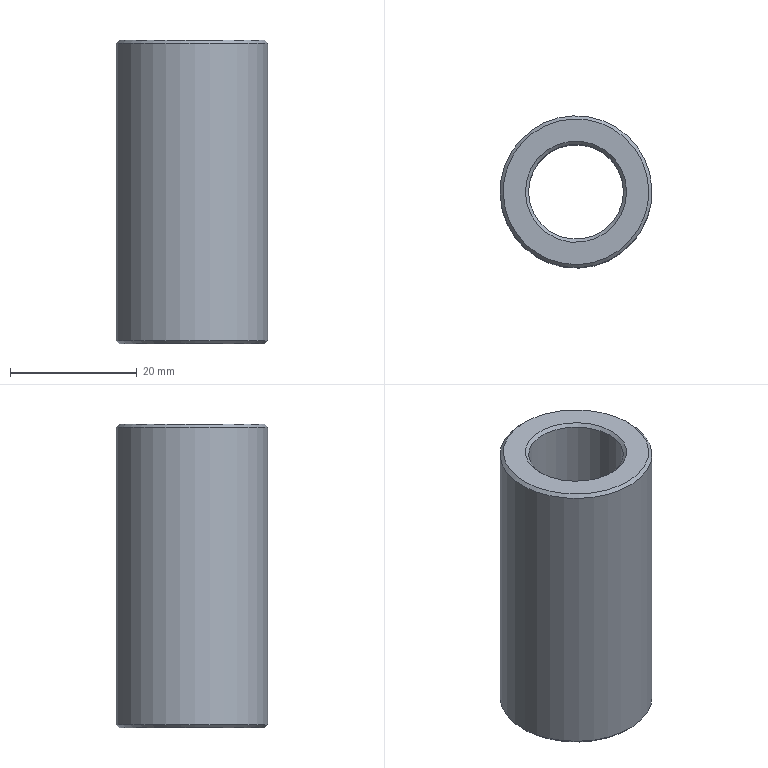Component | NX | BUSHING | 1 solid | 8 faces | box 24 x 24 x 48 mm | volume 13202 mm3 | cone 4 | cylinder 2 | plane 2 | commonest cylinder face diameters 24 x1 15 x1
STEP:
#1=CARTESIAN_POINT('',(0.,0.,0.));
#2=DIRECTION('',(0.,0.,1.));
#3=DIRECTION('',(1.,0.,0.));
#4=AXIS2_PLACEMENT_3D('',#1,#2,#3);
#5=CARTESIAN_POINT('',(-39.104,-11.276,75.5));
#6=VERTEX_POINT('',#5);
#7=CARTESIAN_POINT('',(-35.,0.,75.5));
#8=DIRECTION('',(0.,0.,1.));
#9=DIRECTION('',(-0.342,-0.9397,0.));
#10=AXIS2_PLACEMENT_3D('',#7,#8,#9);
#11=CIRCLE('',#10,12.);
#12=CARTESIAN_POINT('',(-35.,0.,123.));
#13=DIRECTION('',(0.,0.,-1.));
#14=DIRECTION('',(-0.342,-0.9397,0.));
#15=AXIS2_PLACEMENT_3D('',#12,#13,#14);
#16=CYLINDRICAL_SURFACE('',#15,12.);
#17=CARTESIAN_POINT('',(6.283,47.5));
#18=DIRECTION('',(-1.,0.));
#19=VECTOR('',#18,1.);
#20=LINE('',#17,#19);
#21=(GEOMETRIC_REPRESENTATION_CONTEXT(2)PARAMETRIC_REPRESENTATION_CONTEXT()REPRESENTATION_CONTEXT('',''));
#22=DEFINITIONAL_REPRESENTATION('',(#20),#21);
#23=PCURVE('',#16,#22);
#24=CARTESIAN_POINT('',(-35.,0.,75.));
#25=DIRECTION('',(0.,0.,1.));
#26=DIRECTION('',(0.342,0.9397,0.));
#27=AXIS2_PLACEMENT_3D('',#24,#25,#26);
#28=CONICAL_SURFACE('',#27,11.5,0.7854);
#29=CARTESIAN_POINT('',(3.142,0.5));
#30=DIRECTION('',(1.,0.));
#31=VECTOR('',#30,1.);
#32=LINE('',#29,#31);
#33=(GEOMETRIC_REPRESENTATION_CONTEXT(2)PARAMETRIC_REPRESENTATION_CONTEXT()REPRESENTATION_CONTEXT('',''));
#34=DEFINITIONAL_REPRESENTATION('',(#32),#33);
#35=PCURVE('',#28,#34);
#36=SURFACE_CURVE('',#11,(#23,#35),.PCURVE_S1.);
#37=EDGE_CURVE('',#6,#6,#36,.T.);
#38=ORIENTED_EDGE('',*,*,#37,.T.);
#39=CARTESIAN_POINT('',(-39.104,-11.276,122.5));
#40=VERTEX_POINT('',#39);
#41=CARTESIAN_POINT('',(-39.104,-11.276,122.5));
#42=CARTESIAN_POINT('',(-39.104,-11.276,75.5));
#43=B_SPLINE_CURVE_WITH_KNOTS('',1,(#41,#42),.UNSPECIFIED.,.F.,.F.,(2,2),(0.5,47.5),.PIECEWISE_BEZIER_KNOTS.);
#44=CARTESIAN_POINT('',(0.,0.));
#45=DIRECTION('',(0.,1.));
#46=VECTOR('',#45,1.);
#47=LINE('',#44,#46);
#48=(GEOMETRIC_REPRESENTATION_CONTEXT(2)PARAMETRIC_REPRESENTATION_CONTEXT()REPRESENTATION_CONTEXT('',''));
#49=DEFINITIONAL_REPRESENTATION('',(#47),#48);
#50=PCURVE('',#16,#49);
#51=CARTESIAN_POINT('',(6.283,0.));
#52=DIRECTION('',(0.,1.));
#53=VECTOR('',#52,1.);
#54=LINE('',#51,#53);
#55=(GEOMETRIC_REPRESENTATION_CONTEXT(2)PARAMETRIC_REPRESENTATION_CONTEXT()REPRESENTATION_CONTEXT('',''));
#56=DEFINITIONAL_REPRESENTATION('',(#54),#55);
#57=PCURVE('',#16,#56);
#58=SEAM_CURVE('',#43,(#50,#57),.PCURVE_S1.);
#59=EDGE_CURVE('',#40,#6,#58,.T.);
#60=ORIENTED_EDGE('',*,*,#59,.F.);
#61=CARTESIAN_POINT('',(-35.,0.,122.5));
#62=DIRECTION('',(0.,0.,-1.));
#63=DIRECTION('',(-0.342,-0.9397,0.));
#64=AXIS2_PLACEMENT_3D('',#61,#62,#63);
#65=CIRCLE('',#64,12.);
#66=CARTESIAN_POINT('',(0.,0.5));
#67=DIRECTION('',(1.,0.));
#68=VECTOR('',#67,1.);
#69=LINE('',#66,#68);
#70=(GEOMETRIC_REPRESENTATION_CONTEXT(2)PARAMETRIC_REPRESENTATION_CONTEXT()REPRESENTATION_CONTEXT('',''));
#71=DEFINITIONAL_REPRESENTATION('',(#69),#70);
#72=PCURVE('',#16,#71);
#73=CARTESIAN_POINT('',(-35.,0.,122.5));
#74=DIRECTION('',(0.,0.,-1.));
#75=DIRECTION('',(-0.342,-0.9397,0.));
#76=AXIS2_PLACEMENT_3D('',#73,#74,#75);
#77=CONICAL_SURFACE('',#76,12.,0.7854);
#78=CARTESIAN_POINT('',(0.,0.));
#79=DIRECTION('',(1.,0.));
#80=VECTOR('',#79,1.);
#81=LINE('',#78,#80);
#82=(GEOMETRIC_REPRESENTATION_CONTEXT(2)PARAMETRIC_REPRESENTATION_CONTEXT()REPRESENTATION_CONTEXT('',''));
#83=DEFINITIONAL_REPRESENTATION('',(#81),#82);
#84=PCURVE('',#77,#83);
#85=SURFACE_CURVE('',#65,(#72,#84),.PCURVE_S1.);
#86=EDGE_CURVE('',#40,#40,#85,.T.);
#87=ORIENTED_EDGE('',*,*,#86,.T.);
#88=ORIENTED_EDGE('',*,*,#59,.T.);
#89=EDGE_LOOP('',(#38,#60,#87,#88));
#90=FACE_BOUND('',#89,.T.);
#91=ADVANCED_FACE('',(#90),#16,.T.);
#92=CARTESIAN_POINT('',(-37.565,-7.048,75.5));
#93=VERTEX_POINT('',#92);
#94=CARTESIAN_POINT('',(-35.,0.,75.5));
#95=DIRECTION('',(0.,0.,-1.));
#96=DIRECTION('',(-0.342,-0.9397,0.));
#97=AXIS2_PLACEMENT_3D('',#94,#95,#96);
#98=CIRCLE('',#97,7.5);
#99=CARTESIAN_POINT('',(-35.,0.,123.));
#100=DIRECTION('',(0.,0.,-1.));
#101=DIRECTION('',(-0.342,-0.9397,0.));
#102=AXIS2_PLACEMENT_3D('',#99,#100,#101);
#103=CYLINDRICAL_SURFACE('',#102,7.5);
#104=CARTESIAN_POINT('',(0.,47.5));
#105=DIRECTION('',(1.,0.));
#106=VECTOR('',#105,1.);
#107=LINE('',#104,#106);
#108=(GEOMETRIC_REPRESENTATION_CONTEXT(2)PARAMETRIC_REPRESENTATION_CONTEXT()REPRESENTATION_CONTEXT('',''));
#109=DEFINITIONAL_REPRESENTATION('',(#107),#108);
#110=PCURVE('',#103,#109);
#111=CARTESIAN_POINT('',(-35.,0.,75.5));
#112=DIRECTION('',(0.,0.,-1.));
#113=DIRECTION('',(-0.342,-0.9397,0.));
#114=AXIS2_PLACEMENT_3D('',#111,#112,#113);
#115=CONICAL_SURFACE('',#114,7.5,0.7854);
#116=CARTESIAN_POINT('',(0.,0.));
#117=DIRECTION('',(1.,0.));
#118=VECTOR('',#117,1.);
#119=LINE('',#116,#118);
#120=(GEOMETRIC_REPRESENTATION_CONTEXT(2)PARAMETRIC_REPRESENTATION_CONTEXT()REPRESENTATION_CONTEXT('',''));
#121=DEFINITIONAL_REPRESENTATION('',(#119),#120);
#122=PCURVE('',#115,#121);
#123=SURFACE_CURVE('',#98,(#110,#122),.PCURVE_S1.);
#124=EDGE_CURVE('',#93,#93,#123,.T.);
#125=ORIENTED_EDGE('',*,*,#124,.F.);
#126=CARTESIAN_POINT('',(-37.565,-7.048,122.5));
#127=VERTEX_POINT('',#126);
#128=CARTESIAN_POINT('',(-37.565,-7.048,122.5));
#129=CARTESIAN_POINT('',(-37.565,-7.048,75.5));
#130=B_SPLINE_CURVE_WITH_KNOTS('',1,(#128,#129),.UNSPECIFIED.,.F.,.F.,(2,2),(0.5,47.5),.PIECEWISE_BEZIER_KNOTS.);
#131=CARTESIAN_POINT('',(0.,0.));
#132=DIRECTION('',(0.,1.));
#133=VECTOR('',#132,1.);
#134=LINE('',#131,#133);
#135=(GEOMETRIC_REPRESENTATION_CONTEXT(2)PARAMETRIC_REPRESENTATION_CONTEXT()REPRESENTATION_CONTEXT('',''));
#136=DEFINITIONAL_REPRESENTATION('',(#134),#135);
#137=PCURVE('',#103,#136);
#138=CARTESIAN_POINT('',(6.283,0.));
#139=DIRECTION('',(0.,1.));
#140=VECTOR('',#139,1.);
#141=LINE('',#138,#140);
#142=(GEOMETRIC_REPRESENTATION_CONTEXT(2)PARAMETRIC_REPRESENTATION_CONTEXT()REPRESENTATION_CONTEXT('',''));
#143=DEFINITIONAL_REPRESENTATION('',(#141),#142);
#144=PCURVE('',#103,#143);
#145=SEAM_CURVE('',#130,(#137,#144),.PCURVE_S1.);
#146=EDGE_CURVE('',#127,#93,#145,.T.);
#147=ORIENTED_EDGE('',*,*,#146,.F.);
#148=CARTESIAN_POINT('',(-35.,0.,122.5));
#149=DIRECTION('',(0.,0.,1.));
#150=DIRECTION('',(-0.342,-0.9397,0.));
#151=AXIS2_PLACEMENT_3D('',#148,#149,#150);
#152=CIRCLE('',#151,7.5);
#153=CARTESIAN_POINT('',(6.283,0.5));
#154=DIRECTION('',(-1.,0.));
#155=VECTOR('',#154,1.);
#156=LINE('',#153,#155);
#157=(GEOMETRIC_REPRESENTATION_CONTEXT(2)PARAMETRIC_REPRESENTATION_CONTEXT()REPRESENTATION_CONTEXT('',''));
#158=DEFINITIONAL_REPRESENTATION('',(#156),#157);
#159=PCURVE('',#103,#158);
#160=CARTESIAN_POINT('',(-35.,0.,123.));
#161=DIRECTION('',(0.,0.,1.));
#162=DIRECTION('',(0.342,0.9397,0.));
#163=AXIS2_PLACEMENT_3D('',#160,#161,#162);
#164=CONICAL_SURFACE('',#163,8.,0.7854);
#165=CARTESIAN_POINT('',(3.142,-0.5));
#166=DIRECTION('',(1.,0.));
#167=VECTOR('',#166,1.);
#168=LINE('',#165,#167);
#169=(GEOMETRIC_REPRESENTATION_CONTEXT(2)PARAMETRIC_REPRESENTATION_CONTEXT()REPRESENTATION_CONTEXT('',''));
#170=DEFINITIONAL_REPRESENTATION('',(#168),#169);
#171=PCURVE('',#164,#170);
#172=SURFACE_CURVE('',#152,(#159,#171),.PCURVE_S1.);
#173=EDGE_CURVE('',#127,#127,#172,.T.);
#174=ORIENTED_EDGE('',*,*,#173,.F.);
#175=ORIENTED_EDGE('',*,*,#146,.T.);
#176=EDGE_LOOP('',(#125,#147,#174,#175));
#177=FACE_BOUND('',#176,.F.);
#178=ADVANCED_FACE('',(#177),#103,.F.);
#179=CARTESIAN_POINT('',(-37.736,-7.518,123.));
#180=VERTEX_POINT('',#179);
#181=CARTESIAN_POINT('',(-35.,0.,123.));
#182=DIRECTION('',(0.,0.,-1.));
#183=DIRECTION('',(-0.342,-0.9397,0.));
#184=AXIS2_PLACEMENT_3D('',#181,#182,#183);
#185=CIRCLE('',#184,8.);
#186=CARTESIAN_POINT('',(-35.,0.,123.));
#187=DIRECTION('',(0.,0.,-1.));
#188=DIRECTION('',(-0.342,-0.9397,0.));
#189=AXIS2_PLACEMENT_3D('',#186,#187,#188);
#190=PLANE('',#189);
#191=CARTESIAN_POINT('',(0.,0.));
#192=DIRECTION('',(1.,0.));
#193=AXIS2_PLACEMENT_2D('',#191,#192);
#194=CIRCLE('',#193,8.);
#195=(GEOMETRIC_REPRESENTATION_CONTEXT(2)PARAMETRIC_REPRESENTATION_CONTEXT()REPRESENTATION_CONTEXT('',''));
#196=DEFINITIONAL_REPRESENTATION('',(#194),#195);
#197=PCURVE('',#190,#196);
#198=CARTESIAN_POINT('',(9.425,0.));
#199=DIRECTION('',(-1.,0.));
#200=VECTOR('',#199,1.);
#201=LINE('',#198,#200);
#202=(GEOMETRIC_REPRESENTATION_CONTEXT(2)PARAMETRIC_REPRESENTATION_CONTEXT()REPRESENTATION_CONTEXT('',''));
#203=DEFINITIONAL_REPRESENTATION('',(#201),#202);
#204=PCURVE('',#164,#203);
#205=SURFACE_CURVE('',#185,(#197,#204),.PCURVE_S1.);
#206=EDGE_CURVE('',#180,#180,#205,.T.);
#207=ORIENTED_EDGE('',*,*,#206,.T.);
#208=EDGE_LOOP('',(#207));
#209=FACE_BOUND('',#208,.T.);
#210=CARTESIAN_POINT('',(-38.933,-10.806,123.));
#211=VERTEX_POINT('',#210);
#212=CARTESIAN_POINT('',(-35.,0.,123.));
#213=DIRECTION('',(0.,0.,1.));
#214=DIRECTION('',(-0.342,-0.9397,0.));
#215=AXIS2_PLACEMENT_3D('',#212,#213,#214);
#216=CIRCLE('',#215,11.5);
#217=CARTESIAN_POINT('',(11.5,0.));
#218=CARTESIAN_POINT('',(11.5,-19.919));
#219=CARTESIAN_POINT('',(-5.75,-9.959));
#220=CARTESIAN_POINT('',(-23.,-0.));
#221=CARTESIAN_POINT('',(-5.75,9.959));
#222=CARTESIAN_POINT('',(11.5,19.919));
#223=CARTESIAN_POINT('',(11.5,0.));
#224=(BOUNDED_CURVE()B_SPLINE_CURVE(2,(#217,#218,#219,#220,#221,#222,#223),.UNSPECIFIED.,.T.,.F.)B_SPLINE_CURVE_WITH_KNOTS((1,2,2,2,2,1),(-2.094,0.,2.094,4.189,6.283,8.378),.UNSPECIFIED.)CURVE()GEOMETRIC_REPRESENTATION_ITEM()RATIONAL_B_SPLINE_CURVE((1.,0.5,1.,0.5,1.,0.5,1.))REPRESENTATION_ITEM(''));
#225=(GEOMETRIC_REPRESENTATION_CONTEXT(2)PARAMETRIC_REPRESENTATION_CONTEXT()REPRESENTATION_CONTEXT('',''));
#226=DEFINITIONAL_REPRESENTATION('',(#224),#225);
#227=PCURVE('',#190,#226);
#228=CARTESIAN_POINT('',(6.283,-0.5));
#229=DIRECTION('',(-1.,0.));
#230=VECTOR('',#229,1.);
#231=LINE('',#228,#230);
#232=(GEOMETRIC_REPRESENTATION_CONTEXT(2)PARAMETRIC_REPRESENTATION_CONTEXT()REPRESENTATION_CONTEXT('',''));
#233=DEFINITIONAL_REPRESENTATION('',(#231),#232);
#234=PCURVE('',#77,#233);
#235=SURFACE_CURVE('',#216,(#227,#234),.PCURVE_S1.);
#236=EDGE_CURVE('',#211,#211,#235,.T.);
#237=ORIENTED_EDGE('',*,*,#236,.T.);
#238=EDGE_LOOP('',(#237));
#239=FACE_BOUND('',#238,.T.);
#240=ADVANCED_FACE('',(#209,#239),#190,.F.);
#241=CARTESIAN_POINT('',(-38.933,-10.806,75.));
#242=VERTEX_POINT('',#241);
#243=CARTESIAN_POINT('',(-35.,0.,75.));
#244=DIRECTION('',(0.,0.,-1.));
#245=DIRECTION('',(-0.342,-0.9397,0.));
#246=AXIS2_PLACEMENT_3D('',#243,#244,#245);
#247=CIRCLE('',#246,11.5);
#248=CARTESIAN_POINT('',(-35.,0.,75.));
#249=DIRECTION('',(0.,0.,-1.));
#250=DIRECTION('',(-0.342,-0.9397,0.));
#251=AXIS2_PLACEMENT_3D('',#248,#249,#250);
#252=PLANE('',#251);
#253=CARTESIAN_POINT('',(0.,0.));
#254=DIRECTION('',(1.,0.));
#255=AXIS2_PLACEMENT_2D('',#253,#254);
#256=CIRCLE('',#255,11.5);
#257=(GEOMETRIC_REPRESENTATION_CONTEXT(2)PARAMETRIC_REPRESENTATION_CONTEXT()REPRESENTATION_CONTEXT('',''));
#258=DEFINITIONAL_REPRESENTATION('',(#256),#257);
#259=PCURVE('',#252,#258);
#260=CARTESIAN_POINT('',(9.425,0.));
#261=DIRECTION('',(-1.,0.));
#262=VECTOR('',#261,1.);
#263=LINE('',#260,#262);
#264=(GEOMETRIC_REPRESENTATION_CONTEXT(2)PARAMETRIC_REPRESENTATION_CONTEXT()REPRESENTATION_CONTEXT('',''));
#265=DEFINITIONAL_REPRESENTATION('',(#263),#264);
#266=PCURVE('',#28,#265);
#267=SURFACE_CURVE('',#247,(#259,#266),.PCURVE_S1.);
#268=EDGE_CURVE('',#242,#242,#267,.T.);
#269=ORIENTED_EDGE('',*,*,#268,.T.);
#270=EDGE_LOOP('',(#269));
#271=FACE_BOUND('',#270,.T.);
#272=CARTESIAN_POINT('',(-37.736,-7.518,75.));
#273=VERTEX_POINT('',#272);
#274=CARTESIAN_POINT('',(-35.,0.,75.));
#275=DIRECTION('',(0.,0.,1.));
#276=DIRECTION('',(-0.342,-0.9397,0.));
#277=AXIS2_PLACEMENT_3D('',#274,#275,#276);
#278=CIRCLE('',#277,8.);
#279=CARTESIAN_POINT('',(8.,0.));
#280=CARTESIAN_POINT('',(8.,-13.856));
#281=CARTESIAN_POINT('',(-4.,-6.928));
#282=CARTESIAN_POINT('',(-16.,-0.));
#283=CARTESIAN_POINT('',(-4.,6.928));
#284=CARTESIAN_POINT('',(8.,13.856));
#285=CARTESIAN_POINT('',(8.,0.));
#286=(BOUNDED_CURVE()B_SPLINE_CURVE(2,(#279,#280,#281,#282,#283,#284,#285),.UNSPECIFIED.,.T.,.F.)B_SPLINE_CURVE_WITH_KNOTS((1,2,2,2,2,1),(-2.094,0.,2.094,4.189,6.283,8.378),.UNSPECIFIED.)CURVE()GEOMETRIC_REPRESENTATION_ITEM()RATIONAL_B_SPLINE_CURVE((1.,0.5,1.,0.5,1.,0.5,1.))REPRESENTATION_ITEM(''));
#287=(GEOMETRIC_REPRESENTATION_CONTEXT(2)PARAMETRIC_REPRESENTATION_CONTEXT()REPRESENTATION_CONTEXT('',''));
#288=DEFINITIONAL_REPRESENTATION('',(#286),#287);
#289=PCURVE('',#252,#288);
#290=CARTESIAN_POINT('',(6.283,0.5));
#291=DIRECTION('',(-1.,0.));
#292=VECTOR('',#291,1.);
#293=LINE('',#290,#292);
#294=(GEOMETRIC_REPRESENTATION_CONTEXT(2)PARAMETRIC_REPRESENTATION_CONTEXT()REPRESENTATION_CONTEXT('',''));
#295=DEFINITIONAL_REPRESENTATION('',(#293),#294);
#296=PCURVE('',#115,#295);
#297=SURFACE_CURVE('',#278,(#289,#296),.PCURVE_S1.);
#298=EDGE_CURVE('',#273,#273,#297,.T.);
#299=ORIENTED_EDGE('',*,*,#298,.T.);
#300=EDGE_LOOP('',(#299));
#301=FACE_BOUND('',#300,.T.);
#302=ADVANCED_FACE('',(#271,#301),#252,.T.);
#303=ORIENTED_EDGE('',*,*,#37,.F.);
#304=CARTESIAN_POINT('',(-38.933,-10.806,75.));
#305=CARTESIAN_POINT('',(-39.104,-11.276,75.5));
#306=B_SPLINE_CURVE_WITH_KNOTS('',1,(#304,#305),.UNSPECIFIED.,.F.,.F.,(2,2),(0.,0.7071),.PIECEWISE_BEZIER_KNOTS.);
#307=CARTESIAN_POINT('',(3.142,0.));
#308=DIRECTION('',(0.,1.));
#309=VECTOR('',#308,1.);
#310=LINE('',#307,#309);
#311=(GEOMETRIC_REPRESENTATION_CONTEXT(2)PARAMETRIC_REPRESENTATION_CONTEXT()REPRESENTATION_CONTEXT('',''));
#312=DEFINITIONAL_REPRESENTATION('',(#310),#311);
#313=PCURVE('',#28,#312);
#314=CARTESIAN_POINT('',(9.425,0.));
#315=DIRECTION('',(0.,1.));
#316=VECTOR('',#315,1.);
#317=LINE('',#314,#316);
#318=(GEOMETRIC_REPRESENTATION_CONTEXT(2)PARAMETRIC_REPRESENTATION_CONTEXT()REPRESENTATION_CONTEXT('',''));
#319=DEFINITIONAL_REPRESENTATION('',(#317),#318);
#320=PCURVE('',#28,#319);
#321=SEAM_CURVE('',#306,(#313,#320),.PCURVE_S1.);
#322=EDGE_CURVE('',#242,#6,#321,.T.);
#323=ORIENTED_EDGE('',*,*,#322,.F.);
#324=ORIENTED_EDGE('',*,*,#268,.F.);
#325=ORIENTED_EDGE('',*,*,#322,.T.);
#326=EDGE_LOOP('',(#303,#323,#324,#325));
#327=FACE_BOUND('',#326,.T.);
#328=ADVANCED_FACE('',(#327),#28,.T.);
#329=ORIENTED_EDGE('',*,*,#298,.T.);
#330=CARTESIAN_POINT('',(-37.565,-7.048,75.5));
#331=CARTESIAN_POINT('',(-37.736,-7.518,75.));
#332=B_SPLINE_CURVE_WITH_KNOTS('',1,(#330,#331),.UNSPECIFIED.,.F.,.F.,(2,2),(0.,0.7071),.PIECEWISE_BEZIER_KNOTS.);
#333=CARTESIAN_POINT('',(0.,0.));
#334=DIRECTION('',(0.,1.));
#335=VECTOR('',#334,1.);
#336=LINE('',#333,#335);
#337=(GEOMETRIC_REPRESENTATION_CONTEXT(2)PARAMETRIC_REPRESENTATION_CONTEXT()REPRESENTATION_CONTEXT('',''));
#338=DEFINITIONAL_REPRESENTATION('',(#336),#337);
#339=PCURVE('',#115,#338);
#340=CARTESIAN_POINT('',(6.283,0.));
#341=DIRECTION('',(0.,1.));
#342=VECTOR('',#341,1.);
#343=LINE('',#340,#342);
#344=(GEOMETRIC_REPRESENTATION_CONTEXT(2)PARAMETRIC_REPRESENTATION_CONTEXT()REPRESENTATION_CONTEXT('',''));
#345=DEFINITIONAL_REPRESENTATION('',(#343),#344);
#346=PCURVE('',#115,#345);
#347=SEAM_CURVE('',#332,(#339,#346),.PCURVE_S1.);
#348=EDGE_CURVE('',#93,#273,#347,.T.);
#349=ORIENTED_EDGE('',*,*,#348,.F.);
#350=ORIENTED_EDGE('',*,*,#124,.T.);
#351=ORIENTED_EDGE('',*,*,#348,.T.);
#352=EDGE_LOOP('',(#329,#349,#350,#351));
#353=FACE_BOUND('',#352,.F.);
#354=ADVANCED_FACE('',(#353),#115,.F.);
#355=ORIENTED_EDGE('',*,*,#173,.T.);
#356=CARTESIAN_POINT('',(-37.565,-7.048,122.5));
#357=CARTESIAN_POINT('',(-37.736,-7.518,123.));
#358=B_SPLINE_CURVE_WITH_KNOTS('',1,(#356,#357),.UNSPECIFIED.,.F.,.F.,(2,2),(-0.7071,0.),.PIECEWISE_BEZIER_KNOTS.);
#359=CARTESIAN_POINT('',(9.425,0.));
#360=DIRECTION('',(0.,1.));
#361=VECTOR('',#360,1.);
#362=LINE('',#359,#361);
#363=(GEOMETRIC_REPRESENTATION_CONTEXT(2)PARAMETRIC_REPRESENTATION_CONTEXT()REPRESENTATION_CONTEXT('',''));
#364=DEFINITIONAL_REPRESENTATION('',(#362),#363);
#365=PCURVE('',#164,#364);
#366=CARTESIAN_POINT('',(3.142,0.));
#367=DIRECTION('',(0.,1.));
#368=VECTOR('',#367,1.);
#369=LINE('',#366,#368);
#370=(GEOMETRIC_REPRESENTATION_CONTEXT(2)PARAMETRIC_REPRESENTATION_CONTEXT()REPRESENTATION_CONTEXT('',''));
#371=DEFINITIONAL_REPRESENTATION('',(#369),#370);
#372=PCURVE('',#164,#371);
#373=SEAM_CURVE('',#358,(#365,#372),.PCURVE_S1.);
#374=EDGE_CURVE('',#127,#180,#373,.T.);
#375=ORIENTED_EDGE('',*,*,#374,.T.);
#376=ORIENTED_EDGE('',*,*,#206,.T.);
#377=ORIENTED_EDGE('',*,*,#374,.F.);
#378=EDGE_LOOP('',(#355,#375,#376,#377));
#379=FACE_BOUND('',#378,.F.);
#380=ADVANCED_FACE('',(#379),#164,.F.);
#381=ORIENTED_EDGE('',*,*,#236,.F.);
#382=CARTESIAN_POINT('',(-38.933,-10.806,123.));
#383=CARTESIAN_POINT('',(-39.104,-11.276,122.5));
#384=B_SPLINE_CURVE_WITH_KNOTS('',1,(#382,#383),.UNSPECIFIED.,.F.,.F.,(2,2),(-0.7071,0.),.PIECEWISE_BEZIER_KNOTS.);
#385=CARTESIAN_POINT('',(6.283,0.));
#386=DIRECTION('',(0.,1.));
#387=VECTOR('',#386,1.);
#388=LINE('',#385,#387);
#389=(GEOMETRIC_REPRESENTATION_CONTEXT(2)PARAMETRIC_REPRESENTATION_CONTEXT()REPRESENTATION_CONTEXT('',''));
#390=DEFINITIONAL_REPRESENTATION('',(#388),#389);
#391=PCURVE('',#77,#390);
#392=CARTESIAN_POINT('',(0.,0.));
#393=DIRECTION('',(0.,1.));
#394=VECTOR('',#393,1.);
#395=LINE('',#392,#394);
#396=(GEOMETRIC_REPRESENTATION_CONTEXT(2)PARAMETRIC_REPRESENTATION_CONTEXT()REPRESENTATION_CONTEXT('',''));
#397=DEFINITIONAL_REPRESENTATION('',(#395),#396);
#398=PCURVE('',#77,#397);
#399=SEAM_CURVE('',#384,(#391,#398),.PCURVE_S1.);
#400=EDGE_CURVE('',#211,#40,#399,.T.);
#401=ORIENTED_EDGE('',*,*,#400,.T.);
#402=ORIENTED_EDGE('',*,*,#86,.F.);
#403=ORIENTED_EDGE('',*,*,#400,.F.);
#404=EDGE_LOOP('',(#381,#401,#402,#403));
#405=FACE_BOUND('',#404,.T.);
#406=ADVANCED_FACE('',(#405),#77,.T.);
#407=CLOSED_SHELL('',(#91,#178,#240,#302,#328,#354,#380,#406));
#408=MANIFOLD_SOLID_BREP('',#407);
#409=(LENGTH_UNIT()NAMED_UNIT(*)SI_UNIT(.MILLI.,.METRE.));
#410=UNCERTAINTY_MEASURE_WITH_UNIT(LENGTH_MEASURE(0.00001),#409,'','');
#411=(NAMED_UNIT(*)PLANE_ANGLE_UNIT()SI_UNIT($,.RADIAN.));
#412=(NAMED_UNIT(*)SI_UNIT($,.STERADIAN.)SOLID_ANGLE_UNIT());
#413=(GEOMETRIC_REPRESENTATION_CONTEXT(3)GLOBAL_UNCERTAINTY_ASSIGNED_CONTEXT((#410))GLOBAL_UNIT_ASSIGNED_CONTEXT((#409,#411,#412))REPRESENTATION_CONTEXT('',''));
#414=ADVANCED_BREP_SHAPE_REPRESENTATION('',(#4,#408),#413);